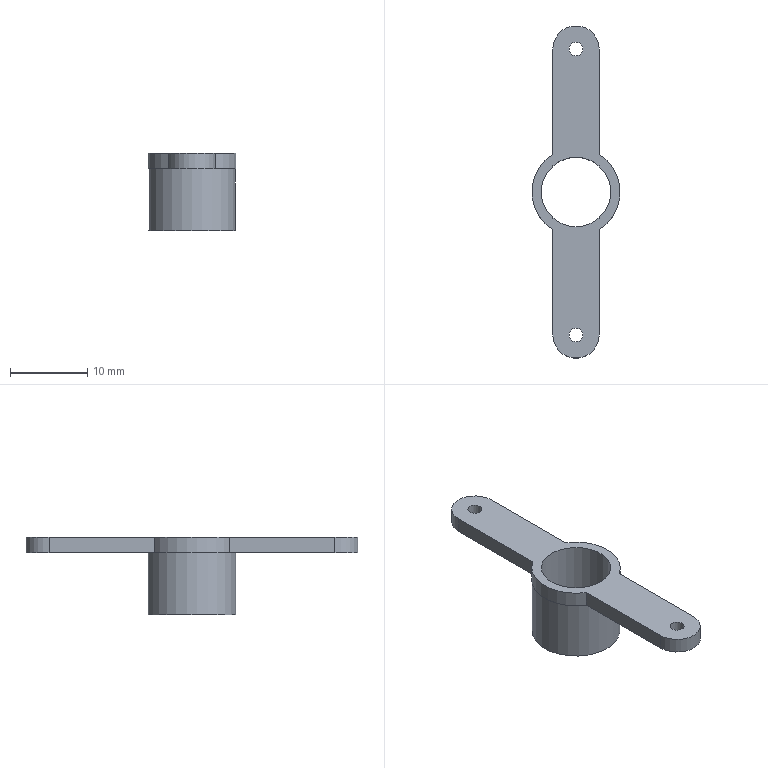Component | NX | MOTOR_MOUNT | 1 solid | 15 faces | box 11.46 x 43 x 10 mm | volume 737 mm3 | cylinder 8 | plane 7 | commonest cylinder face diameters 6 x2 11.458 x2 1.8 x2 9 x1 11.34 x1
STEP:
#1=CARTESIAN_POINT('',(0.,0.,0.));
#2=DIRECTION('',(0.,0.,1.));
#3=DIRECTION('',(1.,0.,0.));
#4=AXIS2_PLACEMENT_3D('',#1,#2,#3);
#5=CARTESIAN_POINT('',(-2.155,-4.204,17.776));
#6=VERTEX_POINT('',#5);
#7=CARTESIAN_POINT('',(-2.155,-17.823,17.776));
#8=VERTEX_POINT('',#7);
#9=CARTESIAN_POINT('',(-2.155,-4.204,17.776));
#10=DIRECTION('',(-0.,-1.,-0.));
#11=VECTOR('',#10,1.);
#12=LINE('',#9,#11);
#13=CARTESIAN_POINT('',(-2.155,-4.204,19.776));
#14=DIRECTION('',(1.,-0.,-0.));
#15=DIRECTION('',(0.,1.,0.));
#16=AXIS2_PLACEMENT_3D('',#13,#14,#15);
#17=PLANE('',#16);
#18=CARTESIAN_POINT('',(0.,-2.));
#19=DIRECTION('',(-1.,-0.));
#20=VECTOR('',#19,1.);
#21=LINE('',#18,#20);
#22=(GEOMETRIC_REPRESENTATION_CONTEXT(2)PARAMETRIC_REPRESENTATION_CONTEXT()REPRESENTATION_CONTEXT('',''));
#23=DEFINITIONAL_REPRESENTATION('',(#21),#22);
#24=PCURVE('',#17,#23);
#25=CARTESIAN_POINT('',(0.8451,-17.823,17.776));
#26=DIRECTION('',(0.,-0.,1.));
#27=DIRECTION('',(0.,-1.,-0.));
#28=AXIS2_PLACEMENT_3D('',#25,#26,#27);
#29=PLANE('',#28);
#30=CARTESIAN_POINT('',(-13.619,-3.));
#31=DIRECTION('',(1.,-0.));
#32=VECTOR('',#31,1.);
#33=LINE('',#30,#32);
#34=(GEOMETRIC_REPRESENTATION_CONTEXT(2)PARAMETRIC_REPRESENTATION_CONTEXT()REPRESENTATION_CONTEXT('',''));
#35=DEFINITIONAL_REPRESENTATION('',(#33),#34);
#36=PCURVE('',#29,#35);
#37=SURFACE_CURVE('',#12,(#24,#36),.PCURVE_S1.);
#38=EDGE_CURVE('',#6,#8,#37,.T.);
#39=ORIENTED_EDGE('',*,*,#38,.T.);
#40=CARTESIAN_POINT('',(-2.155,-17.823,19.776));
#41=VERTEX_POINT('',#40);
#42=CARTESIAN_POINT('',(-2.155,-17.823,19.776));
#43=DIRECTION('',(0.,0.,-1.));
#44=VECTOR('',#43,1.);
#45=LINE('',#42,#44);
#46=CARTESIAN_POINT('',(-13.619,0.));
#47=DIRECTION('',(0.,-1.));
#48=VECTOR('',#47,1.);
#49=LINE('',#46,#48);
#50=(GEOMETRIC_REPRESENTATION_CONTEXT(2)PARAMETRIC_REPRESENTATION_CONTEXT()REPRESENTATION_CONTEXT('',''));
#51=DEFINITIONAL_REPRESENTATION('',(#49),#50);
#52=PCURVE('',#17,#51);
#53=CARTESIAN_POINT('',(0.8451,-17.823,19.776));
#54=DIRECTION('',(0.,0.,-1.));
#55=DIRECTION('',(0.,1.,0.));
#56=AXIS2_PLACEMENT_3D('',#53,#54,#55);
#57=CYLINDRICAL_SURFACE('',#56,3.);
#58=CARTESIAN_POINT('',(4.712,0.));
#59=DIRECTION('',(0.,1.));
#60=VECTOR('',#59,1.);
#61=LINE('',#58,#60);
#62=(GEOMETRIC_REPRESENTATION_CONTEXT(2)PARAMETRIC_REPRESENTATION_CONTEXT()REPRESENTATION_CONTEXT('',''));
#63=DEFINITIONAL_REPRESENTATION('',(#61),#62);
#64=PCURVE('',#57,#63);
#65=SURFACE_CURVE('',#45,(#52,#64),.PCURVE_S1.);
#66=EDGE_CURVE('',#41,#8,#65,.T.);
#67=ORIENTED_EDGE('',*,*,#66,.F.);
#68=CARTESIAN_POINT('',(-2.155,-4.204,19.776));
#69=VERTEX_POINT('',#68);
#70=CARTESIAN_POINT('',(-2.155,-4.204,19.776));
#71=DIRECTION('',(-0.,-1.,-0.));
#72=VECTOR('',#71,1.);
#73=LINE('',#70,#72);
#74=CARTESIAN_POINT('',(0.,0.));
#75=DIRECTION('',(-1.,-0.));
#76=VECTOR('',#75,1.);
#77=LINE('',#74,#76);
#78=(GEOMETRIC_REPRESENTATION_CONTEXT(2)PARAMETRIC_REPRESENTATION_CONTEXT()REPRESENTATION_CONTEXT('',''));
#79=DEFINITIONAL_REPRESENTATION('',(#77),#78);
#80=PCURVE('',#17,#79);
#81=CARTESIAN_POINT('',(0.8451,-17.823,19.776));
#82=DIRECTION('',(0.,-0.,1.));
#83=DIRECTION('',(0.,-1.,-0.));
#84=AXIS2_PLACEMENT_3D('',#81,#82,#83);
#85=PLANE('',#84);
#86=CARTESIAN_POINT('',(-13.619,-3.));
#87=DIRECTION('',(1.,-0.));
#88=VECTOR('',#87,1.);
#89=LINE('',#86,#88);
#90=(GEOMETRIC_REPRESENTATION_CONTEXT(2)PARAMETRIC_REPRESENTATION_CONTEXT()REPRESENTATION_CONTEXT('',''));
#91=DEFINITIONAL_REPRESENTATION('',(#89),#90);
#92=PCURVE('',#85,#91);
#93=SURFACE_CURVE('',#73,(#80,#92),.PCURVE_S1.);
#94=EDGE_CURVE('',#69,#41,#93,.T.);
#95=ORIENTED_EDGE('',*,*,#94,.F.);
#96=CARTESIAN_POINT('',(-2.155,-4.204,19.776));
#97=DIRECTION('',(0.,0.,-1.));
#98=VECTOR('',#97,1.);
#99=LINE('',#96,#98);
#100=CARTESIAN_POINT('',(0.,0.));
#101=DIRECTION('',(0.,-1.));
#102=VECTOR('',#101,1.);
#103=LINE('',#100,#102);
#104=(GEOMETRIC_REPRESENTATION_CONTEXT(2)PARAMETRIC_REPRESENTATION_CONTEXT()REPRESENTATION_CONTEXT('',''));
#105=DEFINITIONAL_REPRESENTATION('',(#103),#104);
#106=PCURVE('',#17,#105);
#107=CARTESIAN_POINT('',(0.8451,0.6765,19.776));
#108=DIRECTION('',(0.,0.,-1.));
#109=DIRECTION('',(0.,1.,0.));
#110=AXIS2_PLACEMENT_3D('',#107,#108,#109);
#111=CYLINDRICAL_SURFACE('',#110,5.729);
#112=CARTESIAN_POINT('',(3.693,-0.));
#113=DIRECTION('',(0.,1.));
#114=VECTOR('',#113,1.);
#115=LINE('',#112,#114);
#116=(GEOMETRIC_REPRESENTATION_CONTEXT(2)PARAMETRIC_REPRESENTATION_CONTEXT()REPRESENTATION_CONTEXT('',''));
#117=DEFINITIONAL_REPRESENTATION('',(#115),#116);
#118=PCURVE('',#111,#117);
#119=SURFACE_CURVE('',#99,(#106,#118),.PCURVE_S1.);
#120=EDGE_CURVE('',#69,#6,#119,.T.);
#121=ORIENTED_EDGE('',*,*,#120,.T.);
#122=EDGE_LOOP('',(#39,#67,#95,#121));
#123=FACE_BOUND('',#122,.T.);
#124=ADVANCED_FACE('',(#123),#17,.F.);
#125=CARTESIAN_POINT('',(3.845,-17.823,17.776));
#126=VERTEX_POINT('',#125);
#127=CARTESIAN_POINT('',(0.8451,-17.823,17.776));
#128=DIRECTION('',(0.,-0.,1.));
#129=DIRECTION('',(0.,-1.,-0.));
#130=AXIS2_PLACEMENT_3D('',#127,#128,#129);
#131=CIRCLE('',#130,3.);
#132=CARTESIAN_POINT('',(9.425,2.));
#133=DIRECTION('',(-1.,0.));
#134=VECTOR('',#133,1.);
#135=LINE('',#132,#134);
#136=(GEOMETRIC_REPRESENTATION_CONTEXT(2)PARAMETRIC_REPRESENTATION_CONTEXT()REPRESENTATION_CONTEXT('',''));
#137=DEFINITIONAL_REPRESENTATION('',(#135),#136);
#138=PCURVE('',#57,#137);
#139=CARTESIAN_POINT('',(0.,0.));
#140=DIRECTION('',(1.,0.));
#141=AXIS2_PLACEMENT_2D('',#139,#140);
#142=CIRCLE('',#141,3.);
#143=(GEOMETRIC_REPRESENTATION_CONTEXT(2)PARAMETRIC_REPRESENTATION_CONTEXT()REPRESENTATION_CONTEXT('',''));
#144=DEFINITIONAL_REPRESENTATION('',(#142),#143);
#145=PCURVE('',#29,#144);
#146=SURFACE_CURVE('',#131,(#138,#145),.PCURVE_S1.);
#147=EDGE_CURVE('',#8,#126,#146,.T.);
#148=ORIENTED_EDGE('',*,*,#147,.T.);
#149=CARTESIAN_POINT('',(3.845,-17.823,19.776));
#150=VERTEX_POINT('',#149);
#151=CARTESIAN_POINT('',(3.845,-17.823,19.776));
#152=DIRECTION('',(0.,0.,-1.));
#153=VECTOR('',#152,1.);
#154=LINE('',#151,#153);
#155=CARTESIAN_POINT('',(1.571,0.));
#156=DIRECTION('',(0.,1.));
#157=VECTOR('',#156,1.);
#158=LINE('',#155,#157);
#159=(GEOMETRIC_REPRESENTATION_CONTEXT(2)PARAMETRIC_REPRESENTATION_CONTEXT()REPRESENTATION_CONTEXT('',''));
#160=DEFINITIONAL_REPRESENTATION('',(#158),#159);
#161=PCURVE('',#57,#160);
#162=CARTESIAN_POINT('',(3.845,-17.823,19.776));
#163=DIRECTION('',(-1.,0.,0.));
#164=DIRECTION('',(-0.,-1.,-0.));
#165=AXIS2_PLACEMENT_3D('',#162,#163,#164);
#166=PLANE('',#165);
#167=CARTESIAN_POINT('',(0.,0.));
#168=DIRECTION('',(-0.,-1.));
#169=VECTOR('',#168,1.);
#170=LINE('',#167,#169);
#171=(GEOMETRIC_REPRESENTATION_CONTEXT(2)PARAMETRIC_REPRESENTATION_CONTEXT()REPRESENTATION_CONTEXT('',''));
#172=DEFINITIONAL_REPRESENTATION('',(#170),#171);
#173=PCURVE('',#166,#172);
#174=SURFACE_CURVE('',#154,(#161,#173),.PCURVE_S1.);
#175=EDGE_CURVE('',#150,#126,#174,.T.);
#176=ORIENTED_EDGE('',*,*,#175,.F.);
#177=CARTESIAN_POINT('',(0.8451,-17.823,19.776));
#178=DIRECTION('',(0.,-0.,1.));
#179=DIRECTION('',(0.,-1.,-0.));
#180=AXIS2_PLACEMENT_3D('',#177,#178,#179);
#181=CIRCLE('',#180,3.);
#182=CARTESIAN_POINT('',(9.425,0.));
#183=DIRECTION('',(-1.,0.));
#184=VECTOR('',#183,1.);
#185=LINE('',#182,#184);
#186=(GEOMETRIC_REPRESENTATION_CONTEXT(2)PARAMETRIC_REPRESENTATION_CONTEXT()REPRESENTATION_CONTEXT('',''));
#187=DEFINITIONAL_REPRESENTATION('',(#185),#186);
#188=PCURVE('',#57,#187);
#189=CARTESIAN_POINT('',(0.,0.));
#190=DIRECTION('',(1.,0.));
#191=AXIS2_PLACEMENT_2D('',#189,#190);
#192=CIRCLE('',#191,3.);
#193=(GEOMETRIC_REPRESENTATION_CONTEXT(2)PARAMETRIC_REPRESENTATION_CONTEXT()REPRESENTATION_CONTEXT('',''));
#194=DEFINITIONAL_REPRESENTATION('',(#192),#193);
#195=PCURVE('',#85,#194);
#196=SURFACE_CURVE('',#181,(#188,#195),.PCURVE_S1.);
#197=EDGE_CURVE('',#41,#150,#196,.T.);
#198=ORIENTED_EDGE('',*,*,#197,.F.);
#199=ORIENTED_EDGE('',*,*,#66,.T.);
#200=EDGE_LOOP('',(#148,#176,#198,#199));
#201=FACE_BOUND('',#200,.T.);
#202=ADVANCED_FACE('',(#201),#57,.T.);
#203=CARTESIAN_POINT('',(3.845,-4.204,17.776));
#204=VERTEX_POINT('',#203);
#205=CARTESIAN_POINT('',(3.845,-17.823,17.776));
#206=DIRECTION('',(0.,1.,0.));
#207=VECTOR('',#206,1.);
#208=LINE('',#205,#207);
#209=CARTESIAN_POINT('',(0.,-2.));
#210=DIRECTION('',(-1.,0.));
#211=VECTOR('',#210,1.);
#212=LINE('',#209,#211);
#213=(GEOMETRIC_REPRESENTATION_CONTEXT(2)PARAMETRIC_REPRESENTATION_CONTEXT()REPRESENTATION_CONTEXT('',''));
#214=DEFINITIONAL_REPRESENTATION('',(#212),#213);
#215=PCURVE('',#166,#214);
#216=CARTESIAN_POINT('',(0.,3.));
#217=DIRECTION('',(-1.,0.));
#218=VECTOR('',#217,1.);
#219=LINE('',#216,#218);
#220=(GEOMETRIC_REPRESENTATION_CONTEXT(2)PARAMETRIC_REPRESENTATION_CONTEXT()REPRESENTATION_CONTEXT('',''));
#221=DEFINITIONAL_REPRESENTATION('',(#219),#220);
#222=PCURVE('',#29,#221);
#223=SURFACE_CURVE('',#208,(#215,#222),.PCURVE_S1.);
#224=EDGE_CURVE('',#126,#204,#223,.T.);
#225=ORIENTED_EDGE('',*,*,#224,.T.);
#226=CARTESIAN_POINT('',(3.845,-4.204,19.776));
#227=VERTEX_POINT('',#226);
#228=CARTESIAN_POINT('',(3.845,-4.204,19.776));
#229=DIRECTION('',(0.,0.,-1.));
#230=VECTOR('',#229,1.);
#231=LINE('',#228,#230);
#232=CARTESIAN_POINT('',(-13.619,-0.));
#233=DIRECTION('',(-0.,-1.));
#234=VECTOR('',#233,1.);
#235=LINE('',#232,#234);
#236=(GEOMETRIC_REPRESENTATION_CONTEXT(2)PARAMETRIC_REPRESENTATION_CONTEXT()REPRESENTATION_CONTEXT('',''));
#237=DEFINITIONAL_REPRESENTATION('',(#235),#236);
#238=PCURVE('',#166,#237);
#239=CARTESIAN_POINT('',(0.8451,0.6765,19.776));
#240=DIRECTION('',(0.,0.,-1.));
#241=DIRECTION('',(0.,1.,0.));
#242=AXIS2_PLACEMENT_3D('',#239,#240,#241);
#243=CYLINDRICAL_SURFACE('',#242,5.729);
#244=CARTESIAN_POINT('',(2.59,-0.));
#245=DIRECTION('',(0.,1.));
#246=VECTOR('',#245,1.);
#247=LINE('',#244,#246);
#248=(GEOMETRIC_REPRESENTATION_CONTEXT(2)PARAMETRIC_REPRESENTATION_CONTEXT()REPRESENTATION_CONTEXT('',''));
#249=DEFINITIONAL_REPRESENTATION('',(#247),#248);
#250=PCURVE('',#243,#249);
#251=SURFACE_CURVE('',#231,(#238,#250),.PCURVE_S1.);
#252=EDGE_CURVE('',#227,#204,#251,.T.);
#253=ORIENTED_EDGE('',*,*,#252,.F.);
#254=CARTESIAN_POINT('',(3.845,-17.823,19.776));
#255=DIRECTION('',(0.,1.,0.));
#256=VECTOR('',#255,1.);
#257=LINE('',#254,#256);
#258=CARTESIAN_POINT('',(0.,0.));
#259=DIRECTION('',(-1.,0.));
#260=VECTOR('',#259,1.);
#261=LINE('',#258,#260);
#262=(GEOMETRIC_REPRESENTATION_CONTEXT(2)PARAMETRIC_REPRESENTATION_CONTEXT()REPRESENTATION_CONTEXT('',''));
#263=DEFINITIONAL_REPRESENTATION('',(#261),#262);
#264=PCURVE('',#166,#263);
#265=CARTESIAN_POINT('',(0.,3.));
#266=DIRECTION('',(-1.,0.));
#267=VECTOR('',#266,1.);
#268=LINE('',#265,#267);
#269=(GEOMETRIC_REPRESENTATION_CONTEXT(2)PARAMETRIC_REPRESENTATION_CONTEXT()REPRESENTATION_CONTEXT('',''));
#270=DEFINITIONAL_REPRESENTATION('',(#268),#269);
#271=PCURVE('',#85,#270);
#272=SURFACE_CURVE('',#257,(#264,#271),.PCURVE_S1.);
#273=EDGE_CURVE('',#150,#227,#272,.T.);
#274=ORIENTED_EDGE('',*,*,#273,.F.);
#275=ORIENTED_EDGE('',*,*,#175,.T.);
#276=EDGE_LOOP('',(#225,#253,#274,#275));
#277=FACE_BOUND('',#276,.T.);
#278=ADVANCED_FACE('',(#277),#166,.F.);
#279=CARTESIAN_POINT('',(3.845,5.557,17.776));
#280=VERTEX_POINT('',#279);
#281=CARTESIAN_POINT('',(0.8451,0.6765,17.776));
#282=DIRECTION('',(0.,-0.,1.));
#283=DIRECTION('',(0.,-1.,-0.));
#284=AXIS2_PLACEMENT_3D('',#281,#282,#283);
#285=CIRCLE('',#284,5.729);
#286=CARTESIAN_POINT('',(3.142,2.));
#287=DIRECTION('',(-1.,0.));
#288=VECTOR('',#287,1.);
#289=LINE('',#286,#288);
#290=(GEOMETRIC_REPRESENTATION_CONTEXT(2)PARAMETRIC_REPRESENTATION_CONTEXT()REPRESENTATION_CONTEXT('',''));
#291=DEFINITIONAL_REPRESENTATION('',(#289),#290);
#292=PCURVE('',#243,#291);
#293=CARTESIAN_POINT('',(-18.5,-0.));
#294=DIRECTION('',(1.,0.));
#295=AXIS2_PLACEMENT_2D('',#293,#294);
#296=CIRCLE('',#295,5.729);
#297=(GEOMETRIC_REPRESENTATION_CONTEXT(2)PARAMETRIC_REPRESENTATION_CONTEXT()REPRESENTATION_CONTEXT('',''));
#298=DEFINITIONAL_REPRESENTATION('',(#296),#297);
#299=PCURVE('',#29,#298);
#300=SURFACE_CURVE('',#285,(#292,#299),.PCURVE_S1.);
#301=EDGE_CURVE('',#204,#280,#300,.T.);
#302=ORIENTED_EDGE('',*,*,#301,.T.);
#303=CARTESIAN_POINT('',(3.845,5.557,19.776));
#304=VERTEX_POINT('',#303);
#305=CARTESIAN_POINT('',(3.845,5.557,19.776));
#306=DIRECTION('',(0.,0.,-1.));
#307=VECTOR('',#306,1.);
#308=LINE('',#305,#307);
#309=CARTESIAN_POINT('',(0.5511,0.));
#310=DIRECTION('',(0.,1.));
#311=VECTOR('',#310,1.);
#312=LINE('',#309,#311);
#313=(GEOMETRIC_REPRESENTATION_CONTEXT(2)PARAMETRIC_REPRESENTATION_CONTEXT()REPRESENTATION_CONTEXT('',''));
#314=DEFINITIONAL_REPRESENTATION('',(#312),#313);
#315=PCURVE('',#243,#314);
#316=CARTESIAN_POINT('',(3.845,5.557,19.776));
#317=DIRECTION('',(-1.,0.,0.));
#318=DIRECTION('',(-0.,-1.,-0.));
#319=AXIS2_PLACEMENT_3D('',#316,#317,#318);
#320=PLANE('',#319);
#321=CARTESIAN_POINT('',(-0.,-0.));
#322=DIRECTION('',(-0.,-1.));
#323=VECTOR('',#322,1.);
#324=LINE('',#321,#323);
#325=(GEOMETRIC_REPRESENTATION_CONTEXT(2)PARAMETRIC_REPRESENTATION_CONTEXT()REPRESENTATION_CONTEXT('',''));
#326=DEFINITIONAL_REPRESENTATION('',(#324),#325);
#327=PCURVE('',#320,#326);
#328=SURFACE_CURVE('',#308,(#315,#327),.PCURVE_S1.);
#329=EDGE_CURVE('',#304,#280,#328,.T.);
#330=ORIENTED_EDGE('',*,*,#329,.F.);
#331=CARTESIAN_POINT('',(0.8451,0.6765,19.776));
#332=DIRECTION('',(0.,-0.,1.));
#333=DIRECTION('',(0.,-1.,-0.));
#334=AXIS2_PLACEMENT_3D('',#331,#332,#333);
#335=CIRCLE('',#334,5.729);
#336=CARTESIAN_POINT('',(3.142,-0.));
#337=DIRECTION('',(-1.,0.));
#338=VECTOR('',#337,1.);
#339=LINE('',#336,#338);
#340=(GEOMETRIC_REPRESENTATION_CONTEXT(2)PARAMETRIC_REPRESENTATION_CONTEXT()REPRESENTATION_CONTEXT('',''));
#341=DEFINITIONAL_REPRESENTATION('',(#339),#340);
#342=PCURVE('',#243,#341);
#343=CARTESIAN_POINT('',(-18.5,-0.));
#344=DIRECTION('',(1.,0.));
#345=AXIS2_PLACEMENT_2D('',#343,#344);
#346=CIRCLE('',#345,5.729);
#347=(GEOMETRIC_REPRESENTATION_CONTEXT(2)PARAMETRIC_REPRESENTATION_CONTEXT()REPRESENTATION_CONTEXT('',''));
#348=DEFINITIONAL_REPRESENTATION('',(#346),#347);
#349=PCURVE('',#85,#348);
#350=SURFACE_CURVE('',#335,(#342,#349),.PCURVE_S1.);
#351=EDGE_CURVE('',#227,#304,#350,.T.);
#352=ORIENTED_EDGE('',*,*,#351,.F.);
#353=ORIENTED_EDGE('',*,*,#252,.T.);
#354=EDGE_LOOP('',(#302,#330,#352,#353));
#355=FACE_BOUND('',#354,.T.);
#356=ADVANCED_FACE('',(#355),#243,.T.);
#357=CARTESIAN_POINT('',(3.845,19.177,17.776));
#358=VERTEX_POINT('',#357);
#359=CARTESIAN_POINT('',(3.845,5.557,17.776));
#360=DIRECTION('',(0.,1.,0.));
#361=VECTOR('',#360,1.);
#362=LINE('',#359,#361);
#363=CARTESIAN_POINT('',(-0.,-2.));
#364=DIRECTION('',(-1.,0.));
#365=VECTOR('',#364,1.);
#366=LINE('',#363,#365);
#367=(GEOMETRIC_REPRESENTATION_CONTEXT(2)PARAMETRIC_REPRESENTATION_CONTEXT()REPRESENTATION_CONTEXT('',''));
#368=DEFINITIONAL_REPRESENTATION('',(#366),#367);
#369=PCURVE('',#320,#368);
#370=CARTESIAN_POINT('',(-23.381,3.));
#371=DIRECTION('',(-1.,0.));
#372=VECTOR('',#371,1.);
#373=LINE('',#370,#372);
#374=(GEOMETRIC_REPRESENTATION_CONTEXT(2)PARAMETRIC_REPRESENTATION_CONTEXT()REPRESENTATION_CONTEXT('',''));
#375=DEFINITIONAL_REPRESENTATION('',(#373),#374);
#376=PCURVE('',#29,#375);
#377=SURFACE_CURVE('',#362,(#369,#376),.PCURVE_S1.);
#378=EDGE_CURVE('',#280,#358,#377,.T.);
#379=ORIENTED_EDGE('',*,*,#378,.T.);
#380=CARTESIAN_POINT('',(3.845,19.177,19.776));
#381=VERTEX_POINT('',#380);
#382=CARTESIAN_POINT('',(3.845,19.177,19.776));
#383=DIRECTION('',(0.,0.,-1.));
#384=VECTOR('',#383,1.);
#385=LINE('',#382,#384);
#386=CARTESIAN_POINT('',(-13.619,0.));
#387=DIRECTION('',(-0.,-1.));
#388=VECTOR('',#387,1.);
#389=LINE('',#386,#388);
#390=(GEOMETRIC_REPRESENTATION_CONTEXT(2)PARAMETRIC_REPRESENTATION_CONTEXT()REPRESENTATION_CONTEXT('',''));
#391=DEFINITIONAL_REPRESENTATION('',(#389),#390);
#392=PCURVE('',#320,#391);
#393=CARTESIAN_POINT('',(0.8451,19.177,19.776));
#394=DIRECTION('',(0.,0.,-1.));
#395=DIRECTION('',(0.,1.,0.));
#396=AXIS2_PLACEMENT_3D('',#393,#394,#395);
#397=CYLINDRICAL_SURFACE('',#396,3.);
#398=CARTESIAN_POINT('',(1.571,0.));
#399=DIRECTION('',(0.,1.));
#400=VECTOR('',#399,1.);
#401=LINE('',#398,#400);
#402=(GEOMETRIC_REPRESENTATION_CONTEXT(2)PARAMETRIC_REPRESENTATION_CONTEXT()REPRESENTATION_CONTEXT('',''));
#403=DEFINITIONAL_REPRESENTATION('',(#401),#402);
#404=PCURVE('',#397,#403);
#405=SURFACE_CURVE('',#385,(#392,#404),.PCURVE_S1.);
#406=EDGE_CURVE('',#381,#358,#405,.T.);
#407=ORIENTED_EDGE('',*,*,#406,.F.);
#408=CARTESIAN_POINT('',(3.845,5.557,19.776));
#409=DIRECTION('',(0.,1.,0.));
#410=VECTOR('',#409,1.);
#411=LINE('',#408,#410);
#412=CARTESIAN_POINT('',(0.,0.));
#413=DIRECTION('',(-1.,0.));
#414=VECTOR('',#413,1.);
#415=LINE('',#412,#414);
#416=(GEOMETRIC_REPRESENTATION_CONTEXT(2)PARAMETRIC_REPRESENTATION_CONTEXT()REPRESENTATION_CONTEXT('',''));
#417=DEFINITIONAL_REPRESENTATION('',(#415),#416);
#418=PCURVE('',#320,#417);
#419=CARTESIAN_POINT('',(-23.381,3.));
#420=DIRECTION('',(-1.,0.));
#421=VECTOR('',#420,1.);
#422=LINE('',#419,#421);
#423=(GEOMETRIC_REPRESENTATION_CONTEXT(2)PARAMETRIC_REPRESENTATION_CONTEXT()REPRESENTATION_CONTEXT('',''));
#424=DEFINITIONAL_REPRESENTATION('',(#422),#423);
#425=PCURVE('',#85,#424);
#426=SURFACE_CURVE('',#411,(#418,#425),.PCURVE_S1.);
#427=EDGE_CURVE('',#304,#381,#426,.T.);
#428=ORIENTED_EDGE('',*,*,#427,.F.);
#429=ORIENTED_EDGE('',*,*,#329,.T.);
#430=EDGE_LOOP('',(#379,#407,#428,#429));
#431=FACE_BOUND('',#430,.T.);
#432=ADVANCED_FACE('',(#431),#320,.F.);
#433=CARTESIAN_POINT('',(-2.155,19.177,17.776));
#434=VERTEX_POINT('',#433);
#435=CARTESIAN_POINT('',(0.8451,19.177,17.776));
#436=DIRECTION('',(0.,-0.,1.));
#437=DIRECTION('',(0.,-1.,-0.));
#438=AXIS2_PLACEMENT_3D('',#435,#436,#437);
#439=CIRCLE('',#438,3.);
#440=CARTESIAN_POINT('',(3.142,2.));
#441=DIRECTION('',(-1.,0.));
#442=VECTOR('',#441,1.);
#443=LINE('',#440,#442);
#444=(GEOMETRIC_REPRESENTATION_CONTEXT(2)PARAMETRIC_REPRESENTATION_CONTEXT()REPRESENTATION_CONTEXT('',''));
#445=DEFINITIONAL_REPRESENTATION('',(#443),#444);
#446=PCURVE('',#397,#445);
#447=CARTESIAN_POINT('',(-37.,0.));
#448=DIRECTION('',(1.,0.));
#449=AXIS2_PLACEMENT_2D('',#447,#448);
#450=CIRCLE('',#449,3.);
#451=(GEOMETRIC_REPRESENTATION_CONTEXT(2)PARAMETRIC_REPRESENTATION_CONTEXT()REPRESENTATION_CONTEXT('',''));
#452=DEFINITIONAL_REPRESENTATION('',(#450),#451);
#453=PCURVE('',#29,#452);
#454=SURFACE_CURVE('',#439,(#446,#453),.PCURVE_S1.);
#455=EDGE_CURVE('',#358,#434,#454,.T.);
#456=ORIENTED_EDGE('',*,*,#455,.T.);
#457=CARTESIAN_POINT('',(-2.155,19.177,19.776));
#458=VERTEX_POINT('',#457);
#459=CARTESIAN_POINT('',(-2.155,19.177,19.776));
#460=DIRECTION('',(0.,0.,-1.));
#461=VECTOR('',#460,1.);
#462=LINE('',#459,#461);
#463=CARTESIAN_POINT('',(-1.571,0.));
#464=DIRECTION('',(0.,1.));
#465=VECTOR('',#464,1.);
#466=LINE('',#463,#465);
#467=(GEOMETRIC_REPRESENTATION_CONTEXT(2)PARAMETRIC_REPRESENTATION_CONTEXT()REPRESENTATION_CONTEXT('',''));
#468=DEFINITIONAL_REPRESENTATION('',(#466),#467);
#469=PCURVE('',#397,#468);
#470=CARTESIAN_POINT('',(-2.155,19.177,19.776));
#471=DIRECTION('',(1.,-0.,-0.));
#472=DIRECTION('',(0.,1.,-0.));
#473=AXIS2_PLACEMENT_3D('',#470,#471,#472);
#474=PLANE('',#473);
#475=CARTESIAN_POINT('',(0.,0.));
#476=DIRECTION('',(0.,-1.));
#477=VECTOR('',#476,1.);
#478=LINE('',#475,#477);
#479=(GEOMETRIC_REPRESENTATION_CONTEXT(2)PARAMETRIC_REPRESENTATION_CONTEXT()REPRESENTATION_CONTEXT('',''));
#480=DEFINITIONAL_REPRESENTATION('',(#478),#479);
#481=PCURVE('',#474,#480);
#482=SURFACE_CURVE('',#462,(#469,#481),.PCURVE_S1.);
#483=EDGE_CURVE('',#458,#434,#482,.T.);
#484=ORIENTED_EDGE('',*,*,#483,.F.);
#485=CARTESIAN_POINT('',(0.8451,19.177,19.776));
#486=DIRECTION('',(0.,-0.,1.));
#487=DIRECTION('',(0.,-1.,-0.));
#488=AXIS2_PLACEMENT_3D('',#485,#486,#487);
#489=CIRCLE('',#488,3.);
#490=CARTESIAN_POINT('',(3.142,0.));
#491=DIRECTION('',(-1.,0.));
#492=VECTOR('',#491,1.);
#493=LINE('',#490,#492);
#494=(GEOMETRIC_REPRESENTATION_CONTEXT(2)PARAMETRIC_REPRESENTATION_CONTEXT()REPRESENTATION_CONTEXT('',''));
#495=DEFINITIONAL_REPRESENTATION('',(#493),#494);
#496=PCURVE('',#397,#495);
#497=CARTESIAN_POINT('',(-37.,0.));
#498=DIRECTION('',(1.,0.));
#499=AXIS2_PLACEMENT_2D('',#497,#498);
#500=CIRCLE('',#499,3.);
#501=(GEOMETRIC_REPRESENTATION_CONTEXT(2)PARAMETRIC_REPRESENTATION_CONTEXT()REPRESENTATION_CONTEXT('',''));
#502=DEFINITIONAL_REPRESENTATION('',(#500),#501);
#503=PCURVE('',#85,#502);
#504=SURFACE_CURVE('',#489,(#496,#503),.PCURVE_S1.);
#505=EDGE_CURVE('',#381,#458,#504,.T.);
#506=ORIENTED_EDGE('',*,*,#505,.F.);
#507=ORIENTED_EDGE('',*,*,#406,.T.);
#508=EDGE_LOOP('',(#456,#484,#506,#507));
#509=FACE_BOUND('',#508,.T.);
#510=ADVANCED_FACE('',(#509),#397,.T.);
#511=CARTESIAN_POINT('',(-2.155,5.557,17.776));
#512=VERTEX_POINT('',#511);
#513=CARTESIAN_POINT('',(-2.155,19.177,17.776));
#514=DIRECTION('',(-0.,-1.,-0.));
#515=VECTOR('',#514,1.);
#516=LINE('',#513,#515);
#517=CARTESIAN_POINT('',(0.,-2.));
#518=DIRECTION('',(-1.,-0.));
#519=VECTOR('',#518,1.);
#520=LINE('',#517,#519);
#521=(GEOMETRIC_REPRESENTATION_CONTEXT(2)PARAMETRIC_REPRESENTATION_CONTEXT()REPRESENTATION_CONTEXT('',''));
#522=DEFINITIONAL_REPRESENTATION('',(#520),#521);
#523=PCURVE('',#474,#522);
#524=CARTESIAN_POINT('',(-37.,-3.));
#525=DIRECTION('',(1.,-0.));
#526=VECTOR('',#525,1.);
#527=LINE('',#524,#526);
#528=(GEOMETRIC_REPRESENTATION_CONTEXT(2)PARAMETRIC_REPRESENTATION_CONTEXT()REPRESENTATION_CONTEXT('',''));
#529=DEFINITIONAL_REPRESENTATION('',(#527),#528);
#530=PCURVE('',#29,#529);
#531=SURFACE_CURVE('',#516,(#523,#530),.PCURVE_S1.);
#532=EDGE_CURVE('',#434,#512,#531,.T.);
#533=ORIENTED_EDGE('',*,*,#532,.T.);
#534=CARTESIAN_POINT('',(-2.155,5.557,19.776));
#535=VERTEX_POINT('',#534);
#536=CARTESIAN_POINT('',(-2.155,5.557,19.776));
#537=DIRECTION('',(0.,0.,-1.));
#538=VECTOR('',#537,1.);
#539=LINE('',#536,#538);
#540=CARTESIAN_POINT('',(-13.619,-0.));
#541=DIRECTION('',(0.,-1.));
#542=VECTOR('',#541,1.);
#543=LINE('',#540,#542);
#544=(GEOMETRIC_REPRESENTATION_CONTEXT(2)PARAMETRIC_REPRESENTATION_CONTEXT()REPRESENTATION_CONTEXT('',''));
#545=DEFINITIONAL_REPRESENTATION('',(#543),#544);
#546=PCURVE('',#474,#545);
#547=CARTESIAN_POINT('',(5.732,0.));
#548=DIRECTION('',(0.,1.));
#549=VECTOR('',#548,1.);
#550=LINE('',#547,#549);
#551=(GEOMETRIC_REPRESENTATION_CONTEXT(2)PARAMETRIC_REPRESENTATION_CONTEXT()REPRESENTATION_CONTEXT('',''));
#552=DEFINITIONAL_REPRESENTATION('',(#550),#551);
#553=PCURVE('',#111,#552);
#554=SURFACE_CURVE('',#539,(#546,#553),.PCURVE_S1.);
#555=EDGE_CURVE('',#535,#512,#554,.T.);
#556=ORIENTED_EDGE('',*,*,#555,.F.);
#557=CARTESIAN_POINT('',(-2.155,19.177,19.776));
#558=DIRECTION('',(-0.,-1.,-0.));
#559=VECTOR('',#558,1.);
#560=LINE('',#557,#559);
#561=CARTESIAN_POINT('',(0.,0.));
#562=DIRECTION('',(-1.,-0.));
#563=VECTOR('',#562,1.);
#564=LINE('',#561,#563);
#565=(GEOMETRIC_REPRESENTATION_CONTEXT(2)PARAMETRIC_REPRESENTATION_CONTEXT()REPRESENTATION_CONTEXT('',''));
#566=DEFINITIONAL_REPRESENTATION('',(#564),#565);
#567=PCURVE('',#474,#566);
#568=CARTESIAN_POINT('',(-37.,-3.));
#569=DIRECTION('',(1.,-0.));
#570=VECTOR('',#569,1.);
#571=LINE('',#568,#570);
#572=(GEOMETRIC_REPRESENTATION_CONTEXT(2)PARAMETRIC_REPRESENTATION_CONTEXT()REPRESENTATION_CONTEXT('',''));
#573=DEFINITIONAL_REPRESENTATION('',(#571),#572);
#574=PCURVE('',#85,#573);
#575=SURFACE_CURVE('',#560,(#567,#574),.PCURVE_S1.);
#576=EDGE_CURVE('',#458,#535,#575,.T.);
#577=ORIENTED_EDGE('',*,*,#576,.F.);
#578=ORIENTED_EDGE('',*,*,#483,.T.);
#579=EDGE_LOOP('',(#533,#556,#577,#578));
#580=FACE_BOUND('',#579,.T.);
#581=ADVANCED_FACE('',(#580),#474,.F.);
#582=CARTESIAN_POINT('',(0.8451,-18.723,19.776));
#583=VERTEX_POINT('',#582);
#584=CARTESIAN_POINT('',(0.8451,-17.823,19.776));
#585=DIRECTION('',(0.,-0.,1.));
#586=DIRECTION('',(0.,-1.,-0.));
#587=AXIS2_PLACEMENT_3D('',#584,#585,#586);
#588=CIRCLE('',#587,0.9);
#589=CARTESIAN_POINT('',(0.8451,-17.823,19.776));
#590=DIRECTION('',(0.,0.,-1.));
#591=DIRECTION('',(0.,1.,0.));
#592=AXIS2_PLACEMENT_3D('',#589,#590,#591);
#593=CYLINDRICAL_SURFACE('',#592,0.9);
#594=CARTESIAN_POINT('',(9.425,0.));
#595=DIRECTION('',(-1.,0.));
#596=VECTOR('',#595,1.);
#597=LINE('',#594,#596);
#598=(GEOMETRIC_REPRESENTATION_CONTEXT(2)PARAMETRIC_REPRESENTATION_CONTEXT()REPRESENTATION_CONTEXT('',''));
#599=DEFINITIONAL_REPRESENTATION('',(#597),#598);
#600=PCURVE('',#593,#599);
#601=CARTESIAN_POINT('',(0.,0.));
#602=DIRECTION('',(1.,0.));
#603=AXIS2_PLACEMENT_2D('',#601,#602);
#604=CIRCLE('',#603,0.9);
#605=(GEOMETRIC_REPRESENTATION_CONTEXT(2)PARAMETRIC_REPRESENTATION_CONTEXT()REPRESENTATION_CONTEXT('',''));
#606=DEFINITIONAL_REPRESENTATION('',(#604),#605);
#607=PCURVE('',#85,#606);
#608=SURFACE_CURVE('',#588,(#600,#607),.PCURVE_S1.);
#609=EDGE_CURVE('',#583,#583,#608,.T.);
#610=ORIENTED_EDGE('',*,*,#609,.F.);
#611=CARTESIAN_POINT('',(0.8451,-18.723,17.776));
#612=VERTEX_POINT('',#611);
#613=CARTESIAN_POINT('',(0.8451,-18.723,19.776));
#614=CARTESIAN_POINT('',(0.8451,-18.723,17.776));
#615=B_SPLINE_CURVE_WITH_KNOTS('',1,(#613,#614),.UNSPECIFIED.,.F.,.F.,(2,2),(0.,2.),.PIECEWISE_BEZIER_KNOTS.);
#616=CARTESIAN_POINT('',(9.425,0.));
#617=DIRECTION('',(0.,1.));
#618=VECTOR('',#617,1.);
#619=LINE('',#616,#618);
#620=(GEOMETRIC_REPRESENTATION_CONTEXT(2)PARAMETRIC_REPRESENTATION_CONTEXT()REPRESENTATION_CONTEXT('',''));
#621=DEFINITIONAL_REPRESENTATION('',(#619),#620);
#622=PCURVE('',#593,#621);
#623=CARTESIAN_POINT('',(3.142,0.));
#624=DIRECTION('',(0.,1.));
#625=VECTOR('',#624,1.);
#626=LINE('',#623,#625);
#627=(GEOMETRIC_REPRESENTATION_CONTEXT(2)PARAMETRIC_REPRESENTATION_CONTEXT()REPRESENTATION_CONTEXT('',''));
#628=DEFINITIONAL_REPRESENTATION('',(#626),#627);
#629=PCURVE('',#593,#628);
#630=SEAM_CURVE('',#615,(#622,#629),.PCURVE_S1.);
#631=EDGE_CURVE('',#583,#612,#630,.T.);
#632=ORIENTED_EDGE('',*,*,#631,.T.);
#633=CARTESIAN_POINT('',(0.8451,-17.823,17.776));
#634=DIRECTION('',(0.,-0.,1.));
#635=DIRECTION('',(0.,-1.,-0.));
#636=AXIS2_PLACEMENT_3D('',#633,#634,#635);
#637=CIRCLE('',#636,0.9);
#638=CARTESIAN_POINT('',(9.425,2.));
#639=DIRECTION('',(-1.,0.));
#640=VECTOR('',#639,1.);
#641=LINE('',#638,#640);
#642=(GEOMETRIC_REPRESENTATION_CONTEXT(2)PARAMETRIC_REPRESENTATION_CONTEXT()REPRESENTATION_CONTEXT('',''));
#643=DEFINITIONAL_REPRESENTATION('',(#641),#642);
#644=PCURVE('',#593,#643);
#645=CARTESIAN_POINT('',(0.,0.));
#646=DIRECTION('',(1.,0.));
#647=AXIS2_PLACEMENT_2D('',#645,#646);
#648=CIRCLE('',#647,0.9);
#649=(GEOMETRIC_REPRESENTATION_CONTEXT(2)PARAMETRIC_REPRESENTATION_CONTEXT()REPRESENTATION_CONTEXT('',''));
#650=DEFINITIONAL_REPRESENTATION('',(#648),#649);
#651=PCURVE('',#29,#650);
#652=SURFACE_CURVE('',#637,(#644,#651),.PCURVE_S1.);
#653=EDGE_CURVE('',#612,#612,#652,.T.);
#654=ORIENTED_EDGE('',*,*,#653,.T.);
#655=ORIENTED_EDGE('',*,*,#631,.F.);
#656=EDGE_LOOP('',(#610,#632,#654,#655));
#657=FACE_BOUND('',#656,.F.);
#658=ADVANCED_FACE('',(#657),#593,.F.);
#659=CARTESIAN_POINT('',(0.8451,-3.823,19.776));
#660=VERTEX_POINT('',#659);
#661=CARTESIAN_POINT('',(0.8451,0.6765,19.776));
#662=DIRECTION('',(0.,-0.,1.));
#663=DIRECTION('',(0.,-1.,-0.));
#664=AXIS2_PLACEMENT_3D('',#661,#662,#663);
#665=CIRCLE('',#664,4.5);
#666=CARTESIAN_POINT('',(0.8451,0.6765,19.776));
#667=DIRECTION('',(0.,0.,-1.));
#668=DIRECTION('',(0.,1.,0.));
#669=AXIS2_PLACEMENT_3D('',#666,#667,#668);
#670=CYLINDRICAL_SURFACE('',#669,4.5);
#671=CARTESIAN_POINT('',(9.425,0.));
#672=DIRECTION('',(-1.,0.));
#673=VECTOR('',#672,1.);
#674=LINE('',#671,#673);
#675=(GEOMETRIC_REPRESENTATION_CONTEXT(2)PARAMETRIC_REPRESENTATION_CONTEXT()REPRESENTATION_CONTEXT('',''));
#676=DEFINITIONAL_REPRESENTATION('',(#674),#675);
#677=PCURVE('',#670,#676);
#678=CARTESIAN_POINT('',(-18.5,-0.));
#679=DIRECTION('',(1.,0.));
#680=AXIS2_PLACEMENT_2D('',#678,#679);
#681=CIRCLE('',#680,4.5);
#682=(GEOMETRIC_REPRESENTATION_CONTEXT(2)PARAMETRIC_REPRESENTATION_CONTEXT()REPRESENTATION_CONTEXT('',''));
#683=DEFINITIONAL_REPRESENTATION('',(#681),#682);
#684=PCURVE('',#85,#683);
#685=SURFACE_CURVE('',#665,(#677,#684),.PCURVE_S1.);
#686=EDGE_CURVE('',#660,#660,#685,.T.);
#687=ORIENTED_EDGE('',*,*,#686,.F.);
#688=CARTESIAN_POINT('',(0.8451,-3.823,9.776));
#689=VERTEX_POINT('',#688);
#690=CARTESIAN_POINT('',(0.8451,-3.823,19.776));
#691=CARTESIAN_POINT('',(0.8451,-3.823,9.776));
#692=B_SPLINE_CURVE_WITH_KNOTS('',1,(#690,#691),.UNSPECIFIED.,.F.,.F.,(2,2),(0.,10.),.PIECEWISE_BEZIER_KNOTS.);
#693=CARTESIAN_POINT('',(9.425,0.));
#694=DIRECTION('',(0.,1.));
#695=VECTOR('',#694,1.);
#696=LINE('',#693,#695);
#697=(GEOMETRIC_REPRESENTATION_CONTEXT(2)PARAMETRIC_REPRESENTATION_CONTEXT()REPRESENTATION_CONTEXT('',''));
#698=DEFINITIONAL_REPRESENTATION('',(#696),#697);
#699=PCURVE('',#670,#698);
#700=CARTESIAN_POINT('',(3.142,0.));
#701=DIRECTION('',(0.,1.));
#702=VECTOR('',#701,1.);
#703=LINE('',#700,#702);
#704=(GEOMETRIC_REPRESENTATION_CONTEXT(2)PARAMETRIC_REPRESENTATION_CONTEXT()REPRESENTATION_CONTEXT('',''));
#705=DEFINITIONAL_REPRESENTATION('',(#703),#704);
#706=PCURVE('',#670,#705);
#707=SEAM_CURVE('',#692,(#699,#706),.PCURVE_S1.);
#708=EDGE_CURVE('',#660,#689,#707,.T.);
#709=ORIENTED_EDGE('',*,*,#708,.T.);
#710=CARTESIAN_POINT('',(0.8451,0.6765,9.776));
#711=DIRECTION('',(-0.,0.,-1.));
#712=DIRECTION('',(0.,-1.,-0.));
#713=AXIS2_PLACEMENT_3D('',#710,#711,#712);
#714=CIRCLE('',#713,4.5);
#715=CARTESIAN_POINT('',(3.142,10.));
#716=DIRECTION('',(1.,0.));
#717=VECTOR('',#716,1.);
#718=LINE('',#715,#717);
#719=(GEOMETRIC_REPRESENTATION_CONTEXT(2)PARAMETRIC_REPRESENTATION_CONTEXT()REPRESENTATION_CONTEXT('',''));
#720=DEFINITIONAL_REPRESENTATION('',(#718),#719);
#721=PCURVE('',#670,#720);
#722=CARTESIAN_POINT('',(0.8451,0.6765,9.776));
#723=DIRECTION('',(0.,-0.,1.));
#724=DIRECTION('',(1.,0.,0.));
#725=AXIS2_PLACEMENT_3D('',#722,#723,#724);
#726=PLANE('',#725);
#727=CARTESIAN_POINT('',(-0.,-4.5));
#728=CARTESIAN_POINT('',(-7.794,-4.5));
#729=CARTESIAN_POINT('',(-3.897,2.25));
#730=CARTESIAN_POINT('',(0.,9.));
#731=CARTESIAN_POINT('',(3.897,2.25));
#732=CARTESIAN_POINT('',(7.794,-4.5));
#733=CARTESIAN_POINT('',(-0.,-4.5));
#734=(BOUNDED_CURVE()B_SPLINE_CURVE(2,(#727,#728,#729,#730,#731,#732,#733),.UNSPECIFIED.,.T.,.F.)B_SPLINE_CURVE_WITH_KNOTS((1,2,2,2,2,1),(-2.094,0.,2.094,4.189,6.283,8.378),.UNSPECIFIED.)CURVE()GEOMETRIC_REPRESENTATION_ITEM()RATIONAL_B_SPLINE_CURVE((1.,0.5,1.,0.5,1.,0.5,1.))REPRESENTATION_ITEM(''));
#735=(GEOMETRIC_REPRESENTATION_CONTEXT(2)PARAMETRIC_REPRESENTATION_CONTEXT()REPRESENTATION_CONTEXT('',''));
#736=DEFINITIONAL_REPRESENTATION('',(#734),#735);
#737=PCURVE('',#726,#736);
#738=SURFACE_CURVE('',#714,(#721,#737),.PCURVE_S1.);
#739=EDGE_CURVE('',#689,#689,#738,.T.);
#740=ORIENTED_EDGE('',*,*,#739,.F.);
#741=ORIENTED_EDGE('',*,*,#708,.F.);
#742=EDGE_LOOP('',(#687,#709,#740,#741));
#743=FACE_BOUND('',#742,.F.);
#744=ADVANCED_FACE('',(#743),#670,.F.);
#745=CARTESIAN_POINT('',(0.8451,0.6765,17.776));
#746=DIRECTION('',(0.,-0.,1.));
#747=DIRECTION('',(0.,-1.,-0.));
#748=AXIS2_PLACEMENT_3D('',#745,#746,#747);
#749=CIRCLE('',#748,5.729);
#750=CARTESIAN_POINT('',(9.425,2.));
#751=DIRECTION('',(-1.,-0.));
#752=VECTOR('',#751,1.);
#753=LINE('',#750,#752);
#754=(GEOMETRIC_REPRESENTATION_CONTEXT(2)PARAMETRIC_REPRESENTATION_CONTEXT()REPRESENTATION_CONTEXT('',''));
#755=DEFINITIONAL_REPRESENTATION('',(#753),#754);
#756=PCURVE('',#111,#755);
#757=CARTESIAN_POINT('',(-18.5,-0.));
#758=DIRECTION('',(1.,0.));
#759=AXIS2_PLACEMENT_2D('',#757,#758);
#760=CIRCLE('',#759,5.729);
#761=(GEOMETRIC_REPRESENTATION_CONTEXT(2)PARAMETRIC_REPRESENTATION_CONTEXT()REPRESENTATION_CONTEXT('',''));
#762=DEFINITIONAL_REPRESENTATION('',(#760),#761);
#763=PCURVE('',#29,#762);
#764=SURFACE_CURVE('',#749,(#756,#763),.PCURVE_S1.);
#765=EDGE_CURVE('',#512,#6,#764,.T.);
#766=ORIENTED_EDGE('',*,*,#765,.T.);
#767=ORIENTED_EDGE('',*,*,#120,.F.);
#768=CARTESIAN_POINT('',(0.8451,0.6765,19.776));
#769=DIRECTION('',(0.,-0.,1.));
#770=DIRECTION('',(0.,-1.,-0.));
#771=AXIS2_PLACEMENT_3D('',#768,#769,#770);
#772=CIRCLE('',#771,5.729);
#773=CARTESIAN_POINT('',(9.425,0.));
#774=DIRECTION('',(-1.,-0.));
#775=VECTOR('',#774,1.);
#776=LINE('',#773,#775);
#777=(GEOMETRIC_REPRESENTATION_CONTEXT(2)PARAMETRIC_REPRESENTATION_CONTEXT()REPRESENTATION_CONTEXT('',''));
#778=DEFINITIONAL_REPRESENTATION('',(#776),#777);
#779=PCURVE('',#111,#778);
#780=CARTESIAN_POINT('',(-18.5,-0.));
#781=DIRECTION('',(1.,0.));
#782=AXIS2_PLACEMENT_2D('',#780,#781);
#783=CIRCLE('',#782,5.729);
#784=(GEOMETRIC_REPRESENTATION_CONTEXT(2)PARAMETRIC_REPRESENTATION_CONTEXT()REPRESENTATION_CONTEXT('',''));
#785=DEFINITIONAL_REPRESENTATION('',(#783),#784);
#786=PCURVE('',#85,#785);
#787=SURFACE_CURVE('',#772,(#779,#786),.PCURVE_S1.);
#788=EDGE_CURVE('',#535,#69,#787,.T.);
#789=ORIENTED_EDGE('',*,*,#788,.F.);
#790=ORIENTED_EDGE('',*,*,#555,.T.);
#791=EDGE_LOOP('',(#766,#767,#789,#790));
#792=FACE_BOUND('',#791,.T.);
#793=ADVANCED_FACE('',(#792),#111,.T.);
#794=CARTESIAN_POINT('',(0.8451,18.277,19.776));
#795=VERTEX_POINT('',#794);
#796=CARTESIAN_POINT('',(0.8451,19.177,19.776));
#797=DIRECTION('',(0.,-0.,1.));
#798=DIRECTION('',(0.,-1.,-0.));
#799=AXIS2_PLACEMENT_3D('',#796,#797,#798);
#800=CIRCLE('',#799,0.9);
#801=CARTESIAN_POINT('',(0.8451,19.177,19.776));
#802=DIRECTION('',(0.,0.,-1.));
#803=DIRECTION('',(0.,1.,0.));
#804=AXIS2_PLACEMENT_3D('',#801,#802,#803);
#805=CYLINDRICAL_SURFACE('',#804,0.9);
#806=CARTESIAN_POINT('',(9.425,0.));
#807=DIRECTION('',(-1.,0.));
#808=VECTOR('',#807,1.);
#809=LINE('',#806,#808);
#810=(GEOMETRIC_REPRESENTATION_CONTEXT(2)PARAMETRIC_REPRESENTATION_CONTEXT()REPRESENTATION_CONTEXT('',''));
#811=DEFINITIONAL_REPRESENTATION('',(#809),#810);
#812=PCURVE('',#805,#811);
#813=CARTESIAN_POINT('',(-37.,0.));
#814=DIRECTION('',(1.,0.));
#815=AXIS2_PLACEMENT_2D('',#813,#814);
#816=CIRCLE('',#815,0.9);
#817=(GEOMETRIC_REPRESENTATION_CONTEXT(2)PARAMETRIC_REPRESENTATION_CONTEXT()REPRESENTATION_CONTEXT('',''));
#818=DEFINITIONAL_REPRESENTATION('',(#816),#817);
#819=PCURVE('',#85,#818);
#820=SURFACE_CURVE('',#800,(#812,#819),.PCURVE_S1.);
#821=EDGE_CURVE('',#795,#795,#820,.T.);
#822=ORIENTED_EDGE('',*,*,#821,.F.);
#823=CARTESIAN_POINT('',(0.8451,18.277,17.776));
#824=VERTEX_POINT('',#823);
#825=CARTESIAN_POINT('',(0.8451,18.277,19.776));
#826=CARTESIAN_POINT('',(0.8451,18.277,17.776));
#827=B_SPLINE_CURVE_WITH_KNOTS('',1,(#825,#826),.UNSPECIFIED.,.F.,.F.,(2,2),(0.,2.),.PIECEWISE_BEZIER_KNOTS.);
#828=CARTESIAN_POINT('',(9.425,0.));
#829=DIRECTION('',(0.,1.));
#830=VECTOR('',#829,1.);
#831=LINE('',#828,#830);
#832=(GEOMETRIC_REPRESENTATION_CONTEXT(2)PARAMETRIC_REPRESENTATION_CONTEXT()REPRESENTATION_CONTEXT('',''));
#833=DEFINITIONAL_REPRESENTATION('',(#831),#832);
#834=PCURVE('',#805,#833);
#835=CARTESIAN_POINT('',(3.142,0.));
#836=DIRECTION('',(0.,1.));
#837=VECTOR('',#836,1.);
#838=LINE('',#835,#837);
#839=(GEOMETRIC_REPRESENTATION_CONTEXT(2)PARAMETRIC_REPRESENTATION_CONTEXT()REPRESENTATION_CONTEXT('',''));
#840=DEFINITIONAL_REPRESENTATION('',(#838),#839);
#841=PCURVE('',#805,#840);
#842=SEAM_CURVE('',#827,(#834,#841),.PCURVE_S1.);
#843=EDGE_CURVE('',#795,#824,#842,.T.);
#844=ORIENTED_EDGE('',*,*,#843,.T.);
#845=CARTESIAN_POINT('',(0.8451,19.177,17.776));
#846=DIRECTION('',(0.,-0.,1.));
#847=DIRECTION('',(0.,-1.,-0.));
#848=AXIS2_PLACEMENT_3D('',#845,#846,#847);
#849=CIRCLE('',#848,0.9);
#850=CARTESIAN_POINT('',(9.425,2.));
#851=DIRECTION('',(-1.,0.));
#852=VECTOR('',#851,1.);
#853=LINE('',#850,#852);
#854=(GEOMETRIC_REPRESENTATION_CONTEXT(2)PARAMETRIC_REPRESENTATION_CONTEXT()REPRESENTATION_CONTEXT('',''));
#855=DEFINITIONAL_REPRESENTATION('',(#853),#854);
#856=PCURVE('',#805,#855);
#857=CARTESIAN_POINT('',(-37.,0.));
#858=DIRECTION('',(1.,0.));
#859=AXIS2_PLACEMENT_2D('',#857,#858);
#860=CIRCLE('',#859,0.9);
#861=(GEOMETRIC_REPRESENTATION_CONTEXT(2)PARAMETRIC_REPRESENTATION_CONTEXT()REPRESENTATION_CONTEXT('',''));
#862=DEFINITIONAL_REPRESENTATION('',(#860),#861);
#863=PCURVE('',#29,#862);
#864=SURFACE_CURVE('',#849,(#856,#863),.PCURVE_S1.);
#865=EDGE_CURVE('',#824,#824,#864,.T.);
#866=ORIENTED_EDGE('',*,*,#865,.T.);
#867=ORIENTED_EDGE('',*,*,#843,.F.);
#868=EDGE_LOOP('',(#822,#844,#866,#867));
#869=FACE_BOUND('',#868,.F.);
#870=ADVANCED_FACE('',(#869),#805,.F.);
#871=ORIENTED_EDGE('',*,*,#94,.T.);
#872=ORIENTED_EDGE('',*,*,#197,.T.);
#873=ORIENTED_EDGE('',*,*,#273,.T.);
#874=ORIENTED_EDGE('',*,*,#351,.T.);
#875=ORIENTED_EDGE('',*,*,#427,.T.);
#876=ORIENTED_EDGE('',*,*,#505,.T.);
#877=ORIENTED_EDGE('',*,*,#576,.T.);
#878=ORIENTED_EDGE('',*,*,#788,.T.);
#879=EDGE_LOOP('',(#871,#872,#873,#874,#875,#876,#877,#878));
#880=FACE_BOUND('',#879,.T.);
#881=ORIENTED_EDGE('',*,*,#686,.F.);
#882=EDGE_LOOP('',(#881));
#883=FACE_BOUND('',#882,.T.);
#884=ORIENTED_EDGE('',*,*,#609,.F.);
#885=EDGE_LOOP('',(#884));
#886=FACE_BOUND('',#885,.T.);
#887=ORIENTED_EDGE('',*,*,#821,.F.);
#888=EDGE_LOOP('',(#887));
#889=FACE_BOUND('',#888,.T.);
#890=ADVANCED_FACE('',(#880,#883,#886,#889),#85,.T.);
#891=CARTESIAN_POINT('',(0.8451,6.347,17.776));
#892=VERTEX_POINT('',#891);
#893=CARTESIAN_POINT('',(0.8451,-4.993,17.776));
#894=VERTEX_POINT('',#893);
#895=CARTESIAN_POINT('',(0.8451,0.6765,17.776));
#896=DIRECTION('',(0.,-0.,1.));
#897=DIRECTION('',(0.,1.,0.));
#898=AXIS2_PLACEMENT_3D('',#895,#896,#897);
#899=CIRCLE('',#898,5.67);
#900=CARTESIAN_POINT('',(-18.5,-0.));
#901=DIRECTION('',(-1.,0.));
#902=AXIS2_PLACEMENT_2D('',#900,#901);
#903=CIRCLE('',#902,5.67);
#904=(GEOMETRIC_REPRESENTATION_CONTEXT(2)PARAMETRIC_REPRESENTATION_CONTEXT()REPRESENTATION_CONTEXT('',''));
#905=DEFINITIONAL_REPRESENTATION('',(#903),#904);
#906=PCURVE('',#29,#905);
#907=CARTESIAN_POINT('',(0.8451,0.6765,-61.424));
#908=DIRECTION('',(0.,-0.,1.));
#909=DIRECTION('',(0.,-1.,-0.));
#910=AXIS2_PLACEMENT_3D('',#907,#908,#909);
#911=CYLINDRICAL_SURFACE('',#910,5.67);
#912=CARTESIAN_POINT('',(3.142,79.2));
#913=DIRECTION('',(1.,0.));
#914=VECTOR('',#913,1.);
#915=LINE('',#912,#914);
#916=(GEOMETRIC_REPRESENTATION_CONTEXT(2)PARAMETRIC_REPRESENTATION_CONTEXT()REPRESENTATION_CONTEXT('',''));
#917=DEFINITIONAL_REPRESENTATION('',(#915),#916);
#918=PCURVE('',#911,#917);
#919=SURFACE_CURVE('',#899,(#906,#918),.PCURVE_S1.);
#920=EDGE_CURVE('',#892,#894,#919,.T.);
#921=ORIENTED_EDGE('',*,*,#920,.T.);
#922=CARTESIAN_POINT('',(0.8451,0.6765,17.776));
#923=DIRECTION('',(0.,-0.,1.));
#924=DIRECTION('',(0.,1.,0.));
#925=AXIS2_PLACEMENT_3D('',#922,#923,#924);
#926=CIRCLE('',#925,5.67);
#927=CARTESIAN_POINT('',(-18.5,-0.));
#928=DIRECTION('',(-1.,0.));
#929=AXIS2_PLACEMENT_2D('',#927,#928);
#930=CIRCLE('',#929,5.67);
#931=(GEOMETRIC_REPRESENTATION_CONTEXT(2)PARAMETRIC_REPRESENTATION_CONTEXT()REPRESENTATION_CONTEXT('',''));
#932=DEFINITIONAL_REPRESENTATION('',(#930),#931);
#933=PCURVE('',#29,#932);
#934=CARTESIAN_POINT('',(-3.142,79.2));
#935=DIRECTION('',(1.,0.));
#936=VECTOR('',#935,1.);
#937=LINE('',#934,#936);
#938=(GEOMETRIC_REPRESENTATION_CONTEXT(2)PARAMETRIC_REPRESENTATION_CONTEXT()REPRESENTATION_CONTEXT('',''));
#939=DEFINITIONAL_REPRESENTATION('',(#937),#938);
#940=PCURVE('',#911,#939);
#941=SURFACE_CURVE('',#926,(#933,#940),.PCURVE_S1.);
#942=EDGE_CURVE('',#894,#892,#941,.T.);
#943=ORIENTED_EDGE('',*,*,#942,.T.);
#944=EDGE_LOOP('',(#921,#943));
#945=FACE_BOUND('',#944,.T.);
#946=ORIENTED_EDGE('',*,*,#38,.F.);
#947=ORIENTED_EDGE('',*,*,#765,.F.);
#948=ORIENTED_EDGE('',*,*,#532,.F.);
#949=ORIENTED_EDGE('',*,*,#455,.F.);
#950=ORIENTED_EDGE('',*,*,#378,.F.);
#951=ORIENTED_EDGE('',*,*,#301,.F.);
#952=ORIENTED_EDGE('',*,*,#224,.F.);
#953=ORIENTED_EDGE('',*,*,#147,.F.);
#954=EDGE_LOOP('',(#946,#947,#948,#949,#950,#951,#952,#953));
#955=FACE_BOUND('',#954,.T.);
#956=ORIENTED_EDGE('',*,*,#653,.T.);
#957=EDGE_LOOP('',(#956));
#958=FACE_BOUND('',#957,.T.);
#959=ORIENTED_EDGE('',*,*,#865,.T.);
#960=EDGE_LOOP('',(#959));
#961=FACE_BOUND('',#960,.T.);
#962=ADVANCED_FACE('',(#945,#955,#958,#961),#29,.F.);
#963=CARTESIAN_POINT('',(0.8451,-4.993,9.776));
#964=VERTEX_POINT('',#963);
#965=CARTESIAN_POINT('',(0.8451,0.6765,9.776));
#966=DIRECTION('',(-0.,0.,-1.));
#967=DIRECTION('',(-0.,-1.,-0.));
#968=AXIS2_PLACEMENT_3D('',#965,#966,#967);
#969=CIRCLE('',#968,5.67);
#970=CARTESIAN_POINT('',(-0.,-5.67));
#971=CARTESIAN_POINT('',(-9.821,-5.67));
#972=CARTESIAN_POINT('',(-4.91,2.835));
#973=CARTESIAN_POINT('',(0.,11.34));
#974=CARTESIAN_POINT('',(4.91,2.835));
#975=CARTESIAN_POINT('',(9.821,-5.67));
#976=CARTESIAN_POINT('',(-0.,-5.67));
#977=(BOUNDED_CURVE()B_SPLINE_CURVE(2,(#970,#971,#972,#973,#974,#975,#976),.UNSPECIFIED.,.T.,.F.)B_SPLINE_CURVE_WITH_KNOTS((1,2,2,2,2,1),(-2.094,0.,2.094,4.189,6.283,8.378),.UNSPECIFIED.)CURVE()GEOMETRIC_REPRESENTATION_ITEM()RATIONAL_B_SPLINE_CURVE((1.,0.5,1.,0.5,1.,0.5,1.))REPRESENTATION_ITEM(''));
#978=(GEOMETRIC_REPRESENTATION_CONTEXT(2)PARAMETRIC_REPRESENTATION_CONTEXT()REPRESENTATION_CONTEXT('',''));
#979=DEFINITIONAL_REPRESENTATION('',(#977),#978);
#980=PCURVE('',#726,#979);
#981=CARTESIAN_POINT('',(6.283,71.2));
#982=DIRECTION('',(-1.,0.));
#983=VECTOR('',#982,1.);
#984=LINE('',#981,#983);
#985=(GEOMETRIC_REPRESENTATION_CONTEXT(2)PARAMETRIC_REPRESENTATION_CONTEXT()REPRESENTATION_CONTEXT('',''));
#986=DEFINITIONAL_REPRESENTATION('',(#984),#985);
#987=PCURVE('',#911,#986);
#988=SURFACE_CURVE('',#969,(#980,#987),.PCURVE_S1.);
#989=EDGE_CURVE('',#964,#964,#988,.T.);
#990=ORIENTED_EDGE('',*,*,#989,.T.);
#991=EDGE_LOOP('',(#990));
#992=FACE_BOUND('',#991,.T.);
#993=ORIENTED_EDGE('',*,*,#739,.F.);
#994=EDGE_LOOP('',(#993));
#995=FACE_BOUND('',#994,.T.);
#996=ADVANCED_FACE('',(#992,#995),#726,.F.);
#997=ORIENTED_EDGE('',*,*,#989,.F.);
#998=CARTESIAN_POINT('',(0.8451,-4.993,9.776));
#999=CARTESIAN_POINT('',(0.8451,-4.993,17.776));
#1000=B_SPLINE_CURVE_WITH_KNOTS('',1,(#998,#999),.UNSPECIFIED.,.F.,.F.,(2,2),(71.2,79.2),.PIECEWISE_BEZIER_KNOTS.);
#1001=CARTESIAN_POINT('',(6.283,0.));
#1002=DIRECTION('',(0.,1.));
#1003=VECTOR('',#1002,1.);
#1004=LINE('',#1001,#1003);
#1005=(GEOMETRIC_REPRESENTATION_CONTEXT(2)PARAMETRIC_REPRESENTATION_CONTEXT()REPRESENTATION_CONTEXT('',''));
#1006=DEFINITIONAL_REPRESENTATION('',(#1004),#1005);
#1007=PCURVE('',#911,#1006);
#1008=CARTESIAN_POINT('',(0.,0.));
#1009=DIRECTION('',(0.,1.));
#1010=VECTOR('',#1009,1.);
#1011=LINE('',#1008,#1010);
#1012=(GEOMETRIC_REPRESENTATION_CONTEXT(2)PARAMETRIC_REPRESENTATION_CONTEXT()REPRESENTATION_CONTEXT('',''));
#1013=DEFINITIONAL_REPRESENTATION('',(#1011),#1012);
#1014=PCURVE('',#911,#1013);
#1015=SEAM_CURVE('',#1000,(#1007,#1014),.PCURVE_S1.);
#1016=EDGE_CURVE('',#964,#894,#1015,.T.);
#1017=ORIENTED_EDGE('',*,*,#1016,.T.);
#1018=ORIENTED_EDGE('',*,*,#920,.F.);
#1019=ORIENTED_EDGE('',*,*,#942,.F.);
#1020=ORIENTED_EDGE('',*,*,#1016,.F.);
#1021=EDGE_LOOP('',(#997,#1017,#1018,#1019,#1020));
#1022=FACE_BOUND('',#1021,.T.);
#1023=ADVANCED_FACE('',(#1022),#911,.T.);
#1024=CLOSED_SHELL('',(#124,#202,#278,#356,#432,#510,#581,#658,#744,#793,#870,#890,#962,#996,#1023));
#1025=MANIFOLD_SOLID_BREP('',#1024);
#1026=(LENGTH_UNIT()NAMED_UNIT(*)SI_UNIT(.MILLI.,.METRE.));
#1027=UNCERTAINTY_MEASURE_WITH_UNIT(LENGTH_MEASURE(0.000002),#1026,'','');
#1028=(NAMED_UNIT(*)PLANE_ANGLE_UNIT()SI_UNIT($,.RADIAN.));
#1029=(NAMED_UNIT(*)SI_UNIT($,.STERADIAN.)SOLID_ANGLE_UNIT());
#1030=(GEOMETRIC_REPRESENTATION_CONTEXT(3)GLOBAL_UNCERTAINTY_ASSIGNED_CONTEXT((#1027))GLOBAL_UNIT_ASSIGNED_CONTEXT((#1026,#1028,#1029))REPRESENTATION_CONTEXT('',''));
#1031=ADVANCED_BREP_SHAPE_REPRESENTATION('',(#4,#1025),#1030);